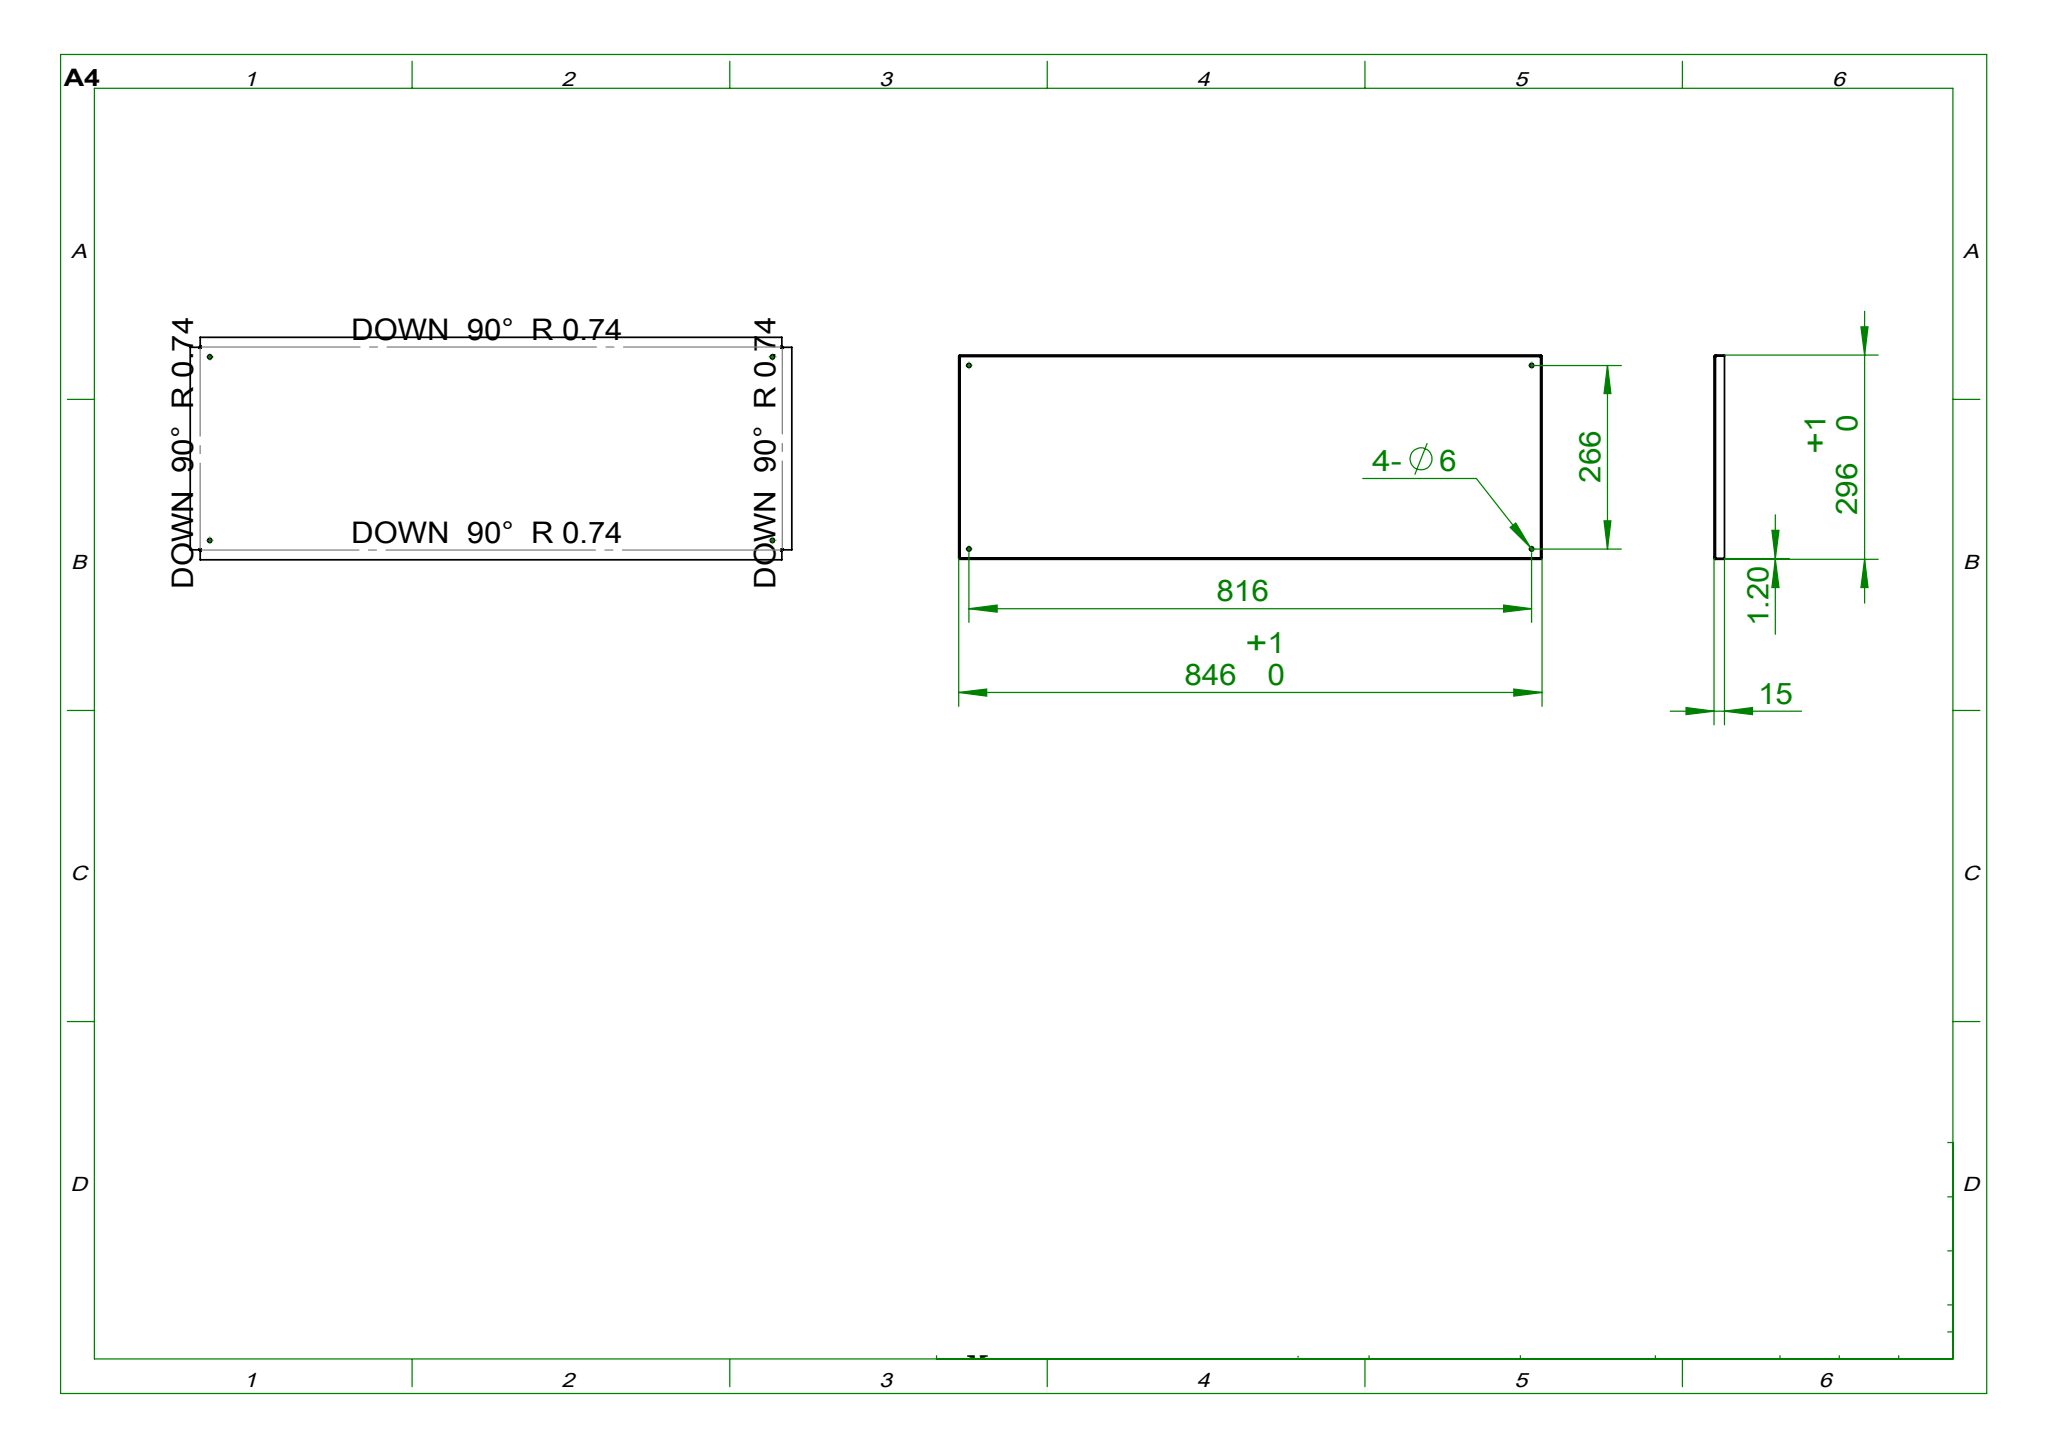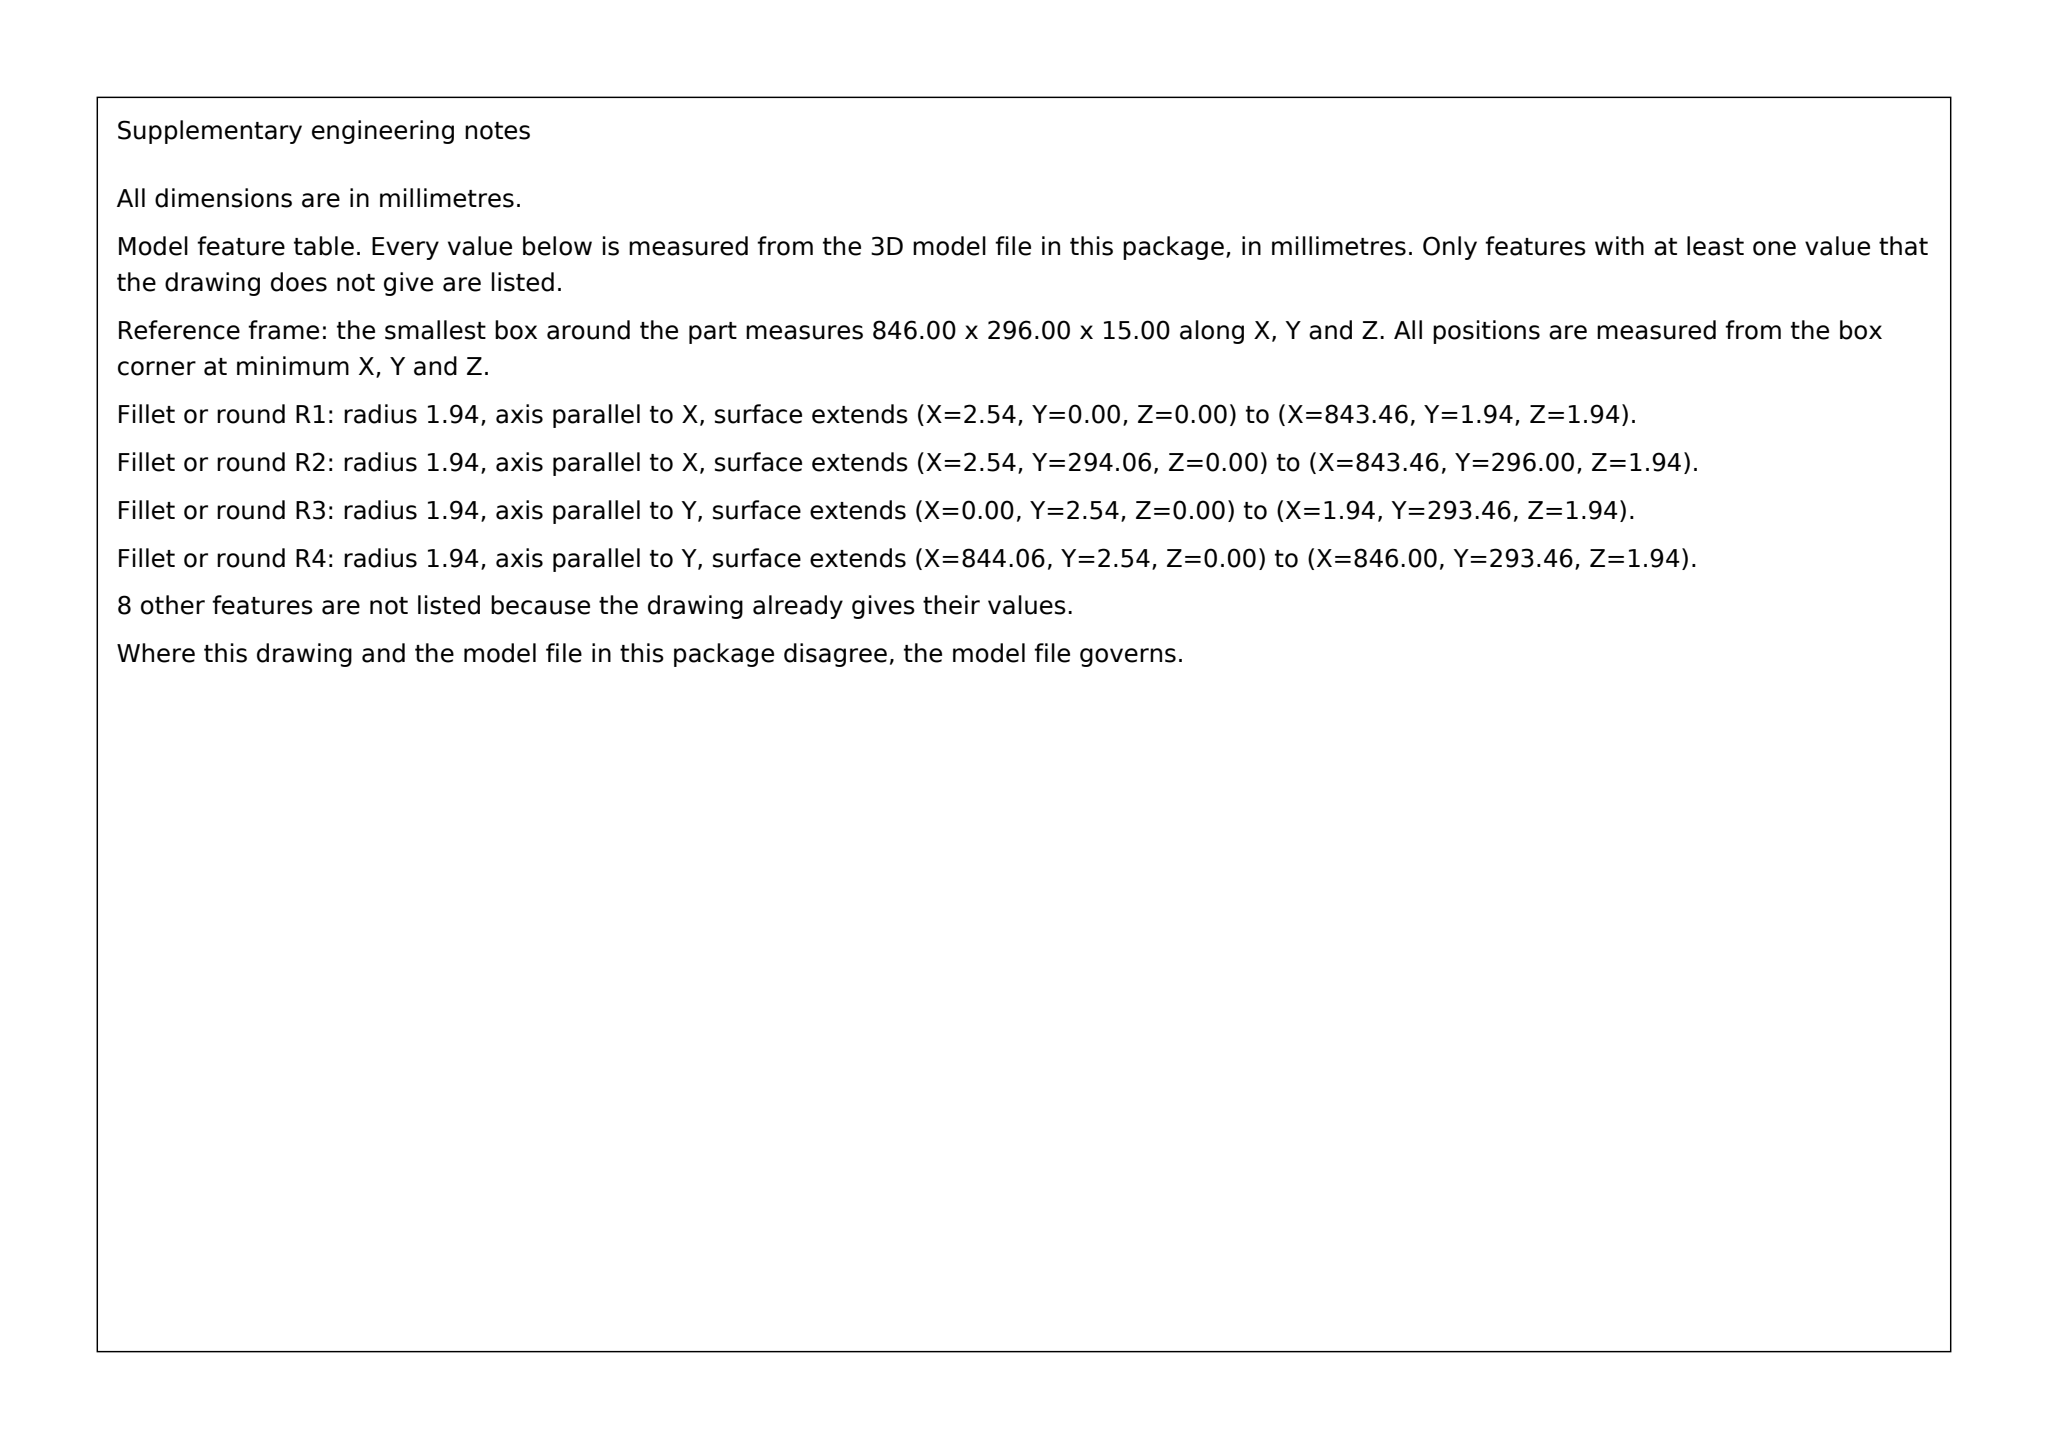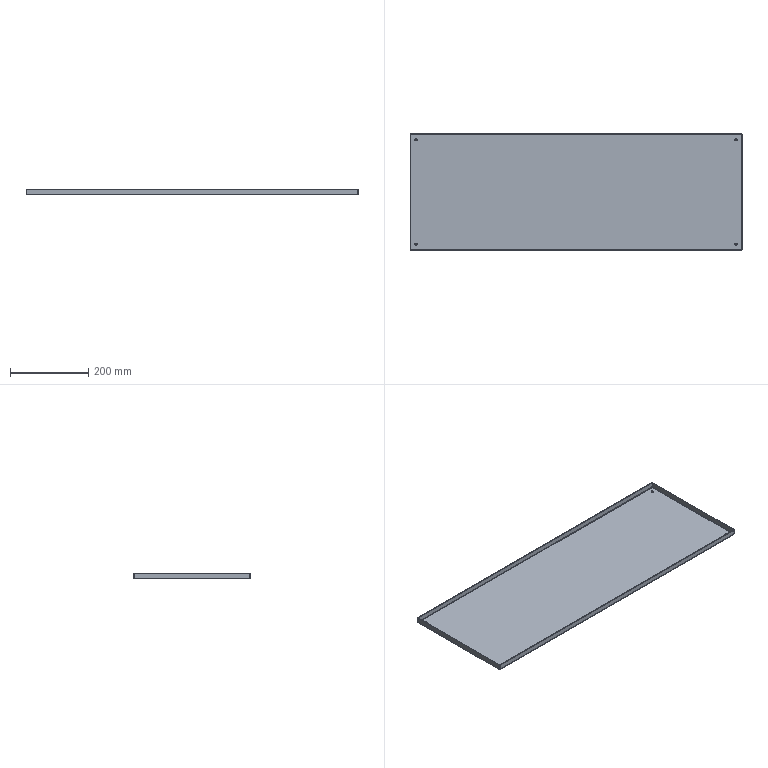Part | SolidWorks | mm | 1 solid | 70 faces | box 846 x 296 x 15 mm | volume 336413 mm3 | plane 54 | cylinder 16 | commonest cylinder face diameters 6 x8 3.873 x4 1.473 x4